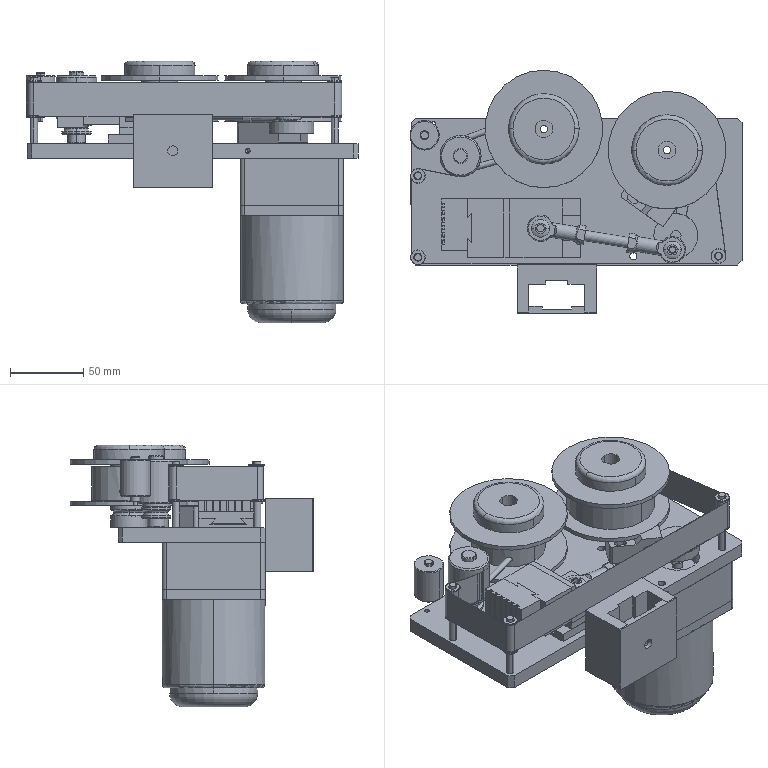Component | SolidWorks | CodingMachine-1 | 32 solids | 747 faces | volume 1069077 mm3 | plane 311 | cylinder 298 | torus 98 | cone 36 | sphere 4 | commonest cylinder face diameters 5 x36 0.4 x36 6 x34 4 x30 10 x23 25 x18 8 x12 12 x10